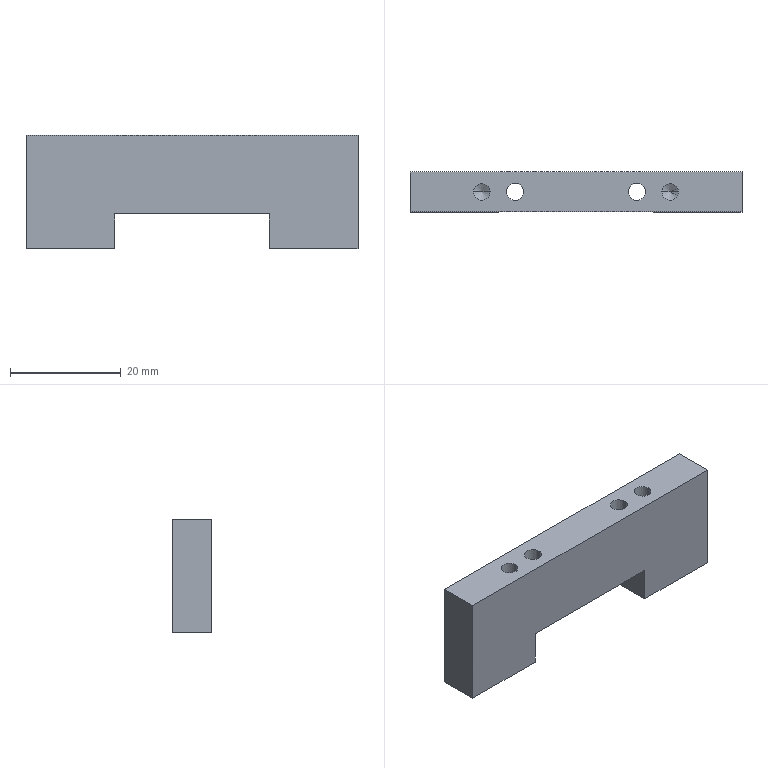Part | SolidWorks | mm | 1 solid | 44 faces | box 60 x 7.2 x 20.5 mm | volume 6969 mm3 | cylinder 20 | cone 12 | plane 12 | commonest cylinder face diameters 3 x8 2.5 x4 5.5 x4 3.1 x4
build123d program:
from build123d import *

# Parameters (mm, degrees)
BOSS_EXTRUDE1_DEPTH                             = 3.6
M3_HEX_SOCKET_HEAD_CAP_SCREW_CBORE1_D           = 3.1
M3_HEX_SOCKET_HEAD_CAP_SCREW_CBORE1_CBORE_D     = 5.5
M3_HEX_SOCKET_HEAD_CAP_SCREW_CBORE1_CBORE_DEPTH = 3.4
M3_TAPPED_HOLE2_D                               = 2.5
M3_TAPPED_HOLE2_DEPTH                           = 8.5
M3_TAPPED_HOLE2_TIP                             = 0.7511
F_3_0_3_DIAMETER_HOLE1_D                        = 3
F_3_0_3_DIAMETER_HOLE1_DEPTH                    = 6
F_3_0_3_DIAMETER_HOLE1_TIP                      = 0.866
F_3_0_3_DIAMETER_HOLE2_D                        = 3
F_3_0_3_DIAMETER_HOLE2_DEPTH                    = 8
F_3_0_3_DIAMETER_HOLE2_TIP                      = 0.866


with BuildPart() as part:
    # Sketch1 → Boss-Extrude1 (new, symmetric)
    with BuildSketch(Plane(origin=(0, 0, 0), x_dir=(1, 0, 0), z_dir=(0, 1, 0))):
        Polygon((-30, 10.25), (-14, 10.25), (-14, 3.95), (14, 3.95), (14, 10.25), (30, 10.25), (30, -10.25), (-30, -10.25), align=None)
    extrude(amount=BOSS_EXTRUDE1_DEPTH, both=True)

    # M3 Hex Socket Head Cap Screw CBORE1 (through all)
    with Locations(Plane(origin=(-3.725, -5.29, -3.95), x_dir=(1, 0, 0), z_dir=(0, 0, -1))):
        with Locations((-7.275, -5.29), (14.725, -5.29)):
            CounterBoreHole(M3_HEX_SOCKET_HEAD_CAP_SCREW_CBORE1_D / 2, M3_HEX_SOCKET_HEAD_CAP_SCREW_CBORE1_CBORE_D / 2, M3_HEX_SOCKET_HEAD_CAP_SCREW_CBORE1_CBORE_DEPTH)

    # M3 Tapped Hole2
    with Locations(Plane(origin=(0, 0, -10.25), x_dir=(-1, 0, 0), z_dir=(0, 0, -1))):
        with Locations((-25, 0), (25, 0)):
            Hole(M3_TAPPED_HOLE2_D / 2, depth=M3_TAPPED_HOLE2_DEPTH)
            with Locations((0, 0, -(M3_TAPPED_HOLE2_DEPTH + M3_TAPPED_HOLE2_TIP / 2))):  # 118° drill point
                Cone(0, M3_TAPPED_HOLE2_D / 2, M3_TAPPED_HOLE2_TIP, mode=Mode.SUBTRACT)

    # 3.0 _3_ Diameter Hole1
    with Locations(Plane(origin=(0, 0, -10.25), x_dir=(-1, 0, 0), z_dir=(0, 0, -1))):
        with Locations((-19, 0), (19, 0)):
            Hole(F_3_0_3_DIAMETER_HOLE1_D / 2, depth=F_3_0_3_DIAMETER_HOLE1_DEPTH)
            with Locations((0, 0, -(F_3_0_3_DIAMETER_HOLE1_DEPTH + F_3_0_3_DIAMETER_HOLE1_TIP / 2))):  # 120° drill point
                Cone(0, F_3_0_3_DIAMETER_HOLE1_D / 2, F_3_0_3_DIAMETER_HOLE1_TIP, mode=Mode.SUBTRACT)

    # 3.0 _3_ Diameter Hole2
    with Locations(Plane.XY.offset(10.25)):
        with Locations((-17, 0), (17, 0)):
            Hole(F_3_0_3_DIAMETER_HOLE2_D / 2, depth=F_3_0_3_DIAMETER_HOLE2_DEPTH)
            with Locations((0, 0, -(F_3_0_3_DIAMETER_HOLE2_DEPTH + F_3_0_3_DIAMETER_HOLE2_TIP / 2))):  # 120° drill point
                Cone(0, F_3_0_3_DIAMETER_HOLE2_D / 2, F_3_0_3_DIAMETER_HOLE2_TIP, mode=Mode.SUBTRACT)


solid = part.part